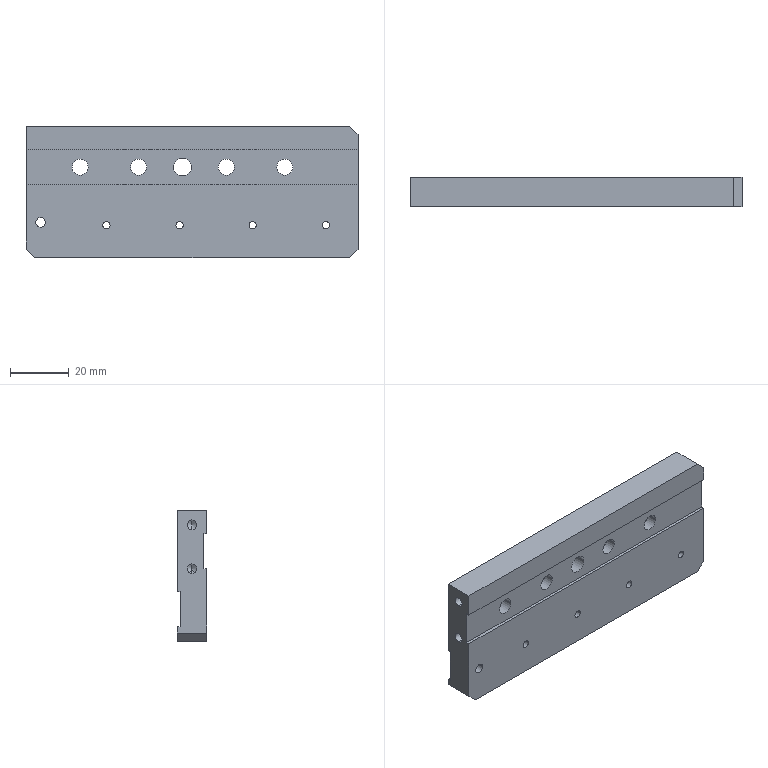Component | SolidWorks | 17268062-1 | 1 solid | 57 faces | box 113.5 x 10 x 45 mm | volume 45407 mm3 | cylinder 32 | plane 21 | cone 4 | commonest cylinder face diameters 10 x8 5.5 x8 2.5 x8 3.3 x6 6 x2 | material SKD-11 HRC58° Hard Chrome Plated
build123d program:
from build123d import *

# Parameters (mm, degrees)
SKETCH1_W                                       = 45
SKETCH1_H                                       = 10
BOSS_EXTRUDE1_DEPTH                             = 113.5
SKETCH2_W                                       = 12
SKETCH2_H                                       = 1
CUT_EXTRUDE1_DEPTH                              = 119.542
M4_TAPPED_HOLE1_D                               = 3.3
M4_TAPPED_HOLE1_DEPTH                           = 15
M4_TAPPED_HOLE1_TIP                             = 0.9914
SKETCH5_W                                       = 12
SKETCH5_H                                       = 1
CUT_EXTRUDE2_DEPTH                              = 119.542
M3_TAPPED_HOLE1_D                               = 2.5
M5_HEX_SOCKET_HEAD_CAP_SCREW_CBORE1_D           = 5.5
M5_HEX_SOCKET_HEAD_CAP_SCREW_CBORE1_CBORE_D     = 10
M5_HEX_SOCKET_HEAD_CAP_SCREW_CBORE1_CBORE_DEPTH = 5.4
CHAMFER1_SIZE                                   = 3
M4_TAPPED_HOLE2_D                               = 3.3
SIZE_MM_DOWEL_PIN_HOLE1_D                       = 6


with BuildPart() as part:
    # Sketch1 → Boss-Extrude1 (new body)
    with BuildSketch(Plane.XY):
        with Locations((-10.5, -4)):
            Rectangle(SKETCH1_W, SKETCH1_H)
    extrude(amount=-BOSS_EXTRUDE1_DEPTH)

    # Sketch2 → Cut-Extrude1 (cut, through all)
    with BuildSketch(Plane.XY):
        with Locations((0.8507, 0.5)):
            Rectangle(SKETCH2_W, SKETCH2_H)
    extrude(amount=-CUT_EXTRUDE1_DEPTH, mode=Mode.SUBTRACT)

    # M4 Tapped Hole1
    with Locations(Plane(origin=(0, 0, -113.5), x_dir=(-1, 0, 0), z_dir=(0, 0, -1))):
        with Locations((13, -4), (28, -4)):
            Hole(M4_TAPPED_HOLE1_D / 2, depth=M4_TAPPED_HOLE1_DEPTH)
            with Locations((0, 0, -(M4_TAPPED_HOLE1_DEPTH + M4_TAPPED_HOLE1_TIP / 2))):  # 118° drill point
                Cone(0, M4_TAPPED_HOLE1_D / 2, M4_TAPPED_HOLE1_TIP, mode=Mode.SUBTRACT)

    # Sketch5 → Cut-Extrude2 (cut, through all)
    with BuildSketch(Plane.XY):
        with Locations((-19, -8.5)):
            Rectangle(SKETCH5_W, SKETCH5_H)
    extrude(amount=-CUT_EXTRUDE2_DEPTH, mode=Mode.SUBTRACT)

    # M3 Tapped Hole1 (through all)
    with Locations(Plane(origin=(0, 0, 0), x_dir=(1, 0, 0), z_dir=(0, 1, 0))):
        with Locations((0.8507, 86), (0.8507, 61), (0.8507, 36), (0.8507, 11)):
            Hole(M3_TAPPED_HOLE1_D / 2)

    # M5 Hex Socket Head Cap Screw CBORE1 (through all)
    with Locations(Plane(origin=(0, 1, 0), x_dir=(1, 0, 0), z_dir=(0, 1, 0))):
        with Locations((-19, 45), (-19, 25), (-19, 75), (-19, 95)):
            CounterBoreHole(M5_HEX_SOCKET_HEAD_CAP_SCREW_CBORE1_D / 2, M5_HEX_SOCKET_HEAD_CAP_SCREW_CBORE1_CBORE_D / 2, M5_HEX_SOCKET_HEAD_CAP_SCREW_CBORE1_CBORE_DEPTH)

    # Chamfer1
    chamfer1_edges = [part.edges().sort_by_distance(p)[0] for p in [
        (12, -4, -113.5),
        (12, -4, 0),
        (-33, -4, 0),
    ]]
    chamfer(chamfer1_edges, length=CHAMFER1_SIZE)

    # M4 Tapped Hole2 (through all)
    with Locations(Plane(origin=(0, 0, 0), x_dir=(1, 0, 0), z_dir=(0, 1, 0))):
        with Locations((-0.1493, 108.5)):
            Hole(M4_TAPPED_HOLE2_D / 2)

    # Size mm Dowel Pin Hole1 (through all)
    with Locations(Plane(origin=(0, 1, 0), x_dir=(1, 0, 0), z_dir=(0, 1, 0))):
        with Locations((-19, 60)):
            Hole(SIZE_MM_DOWEL_PIN_HOLE1_D / 2)


solid = part.part

# Placed as in the assembly
solid = solid.moved(Location((39.5, -43.579, 0.8507), (0, 90, 0)))